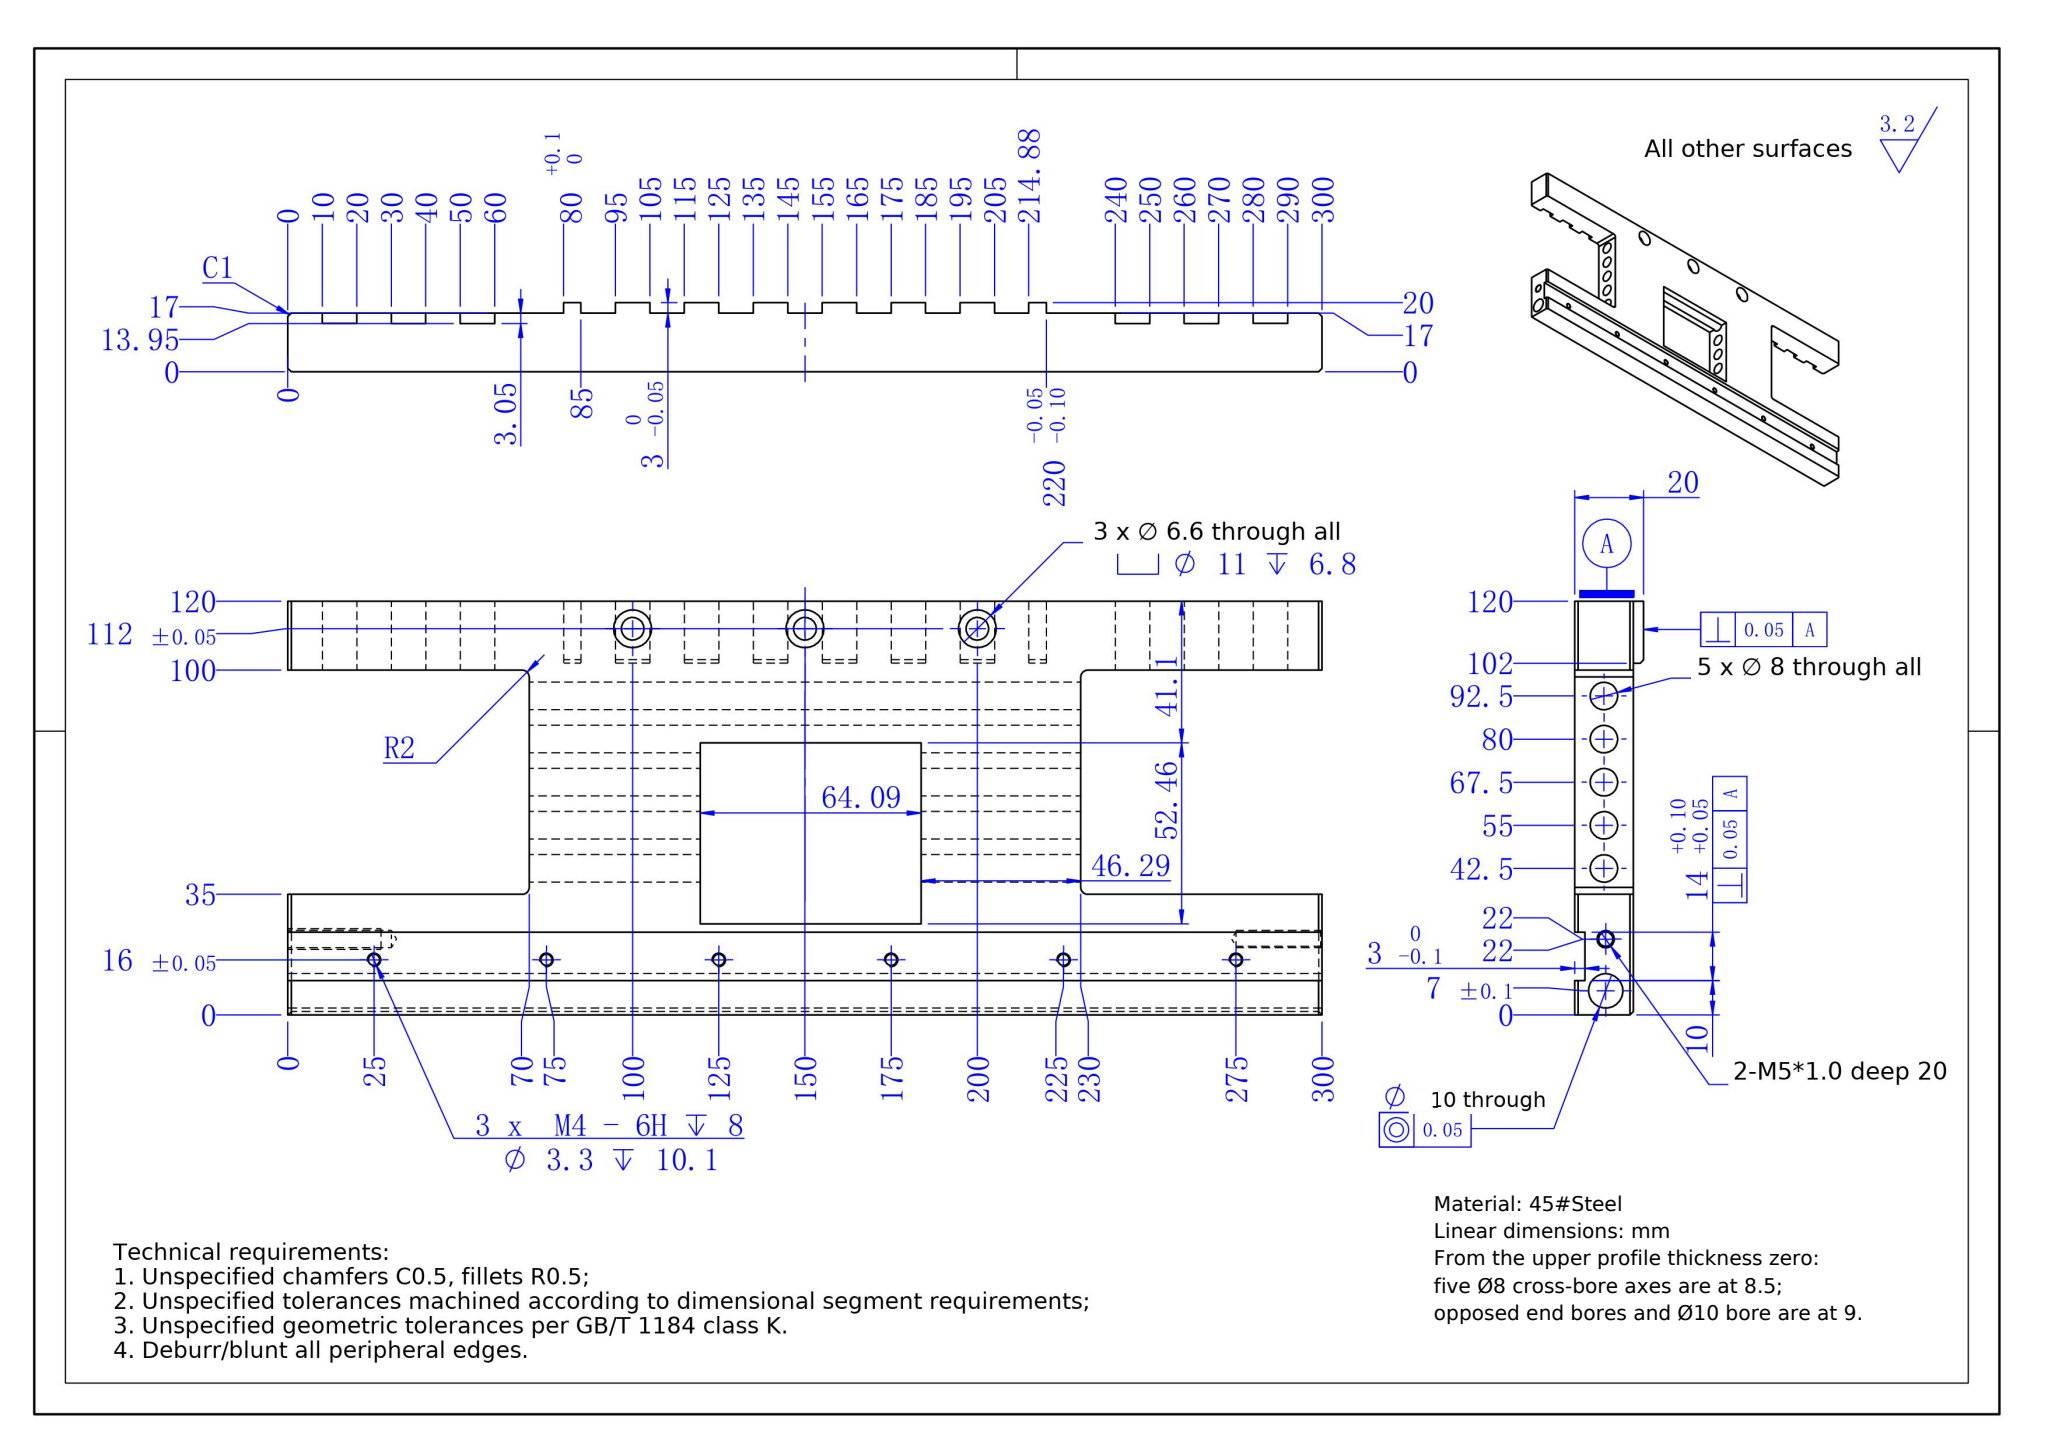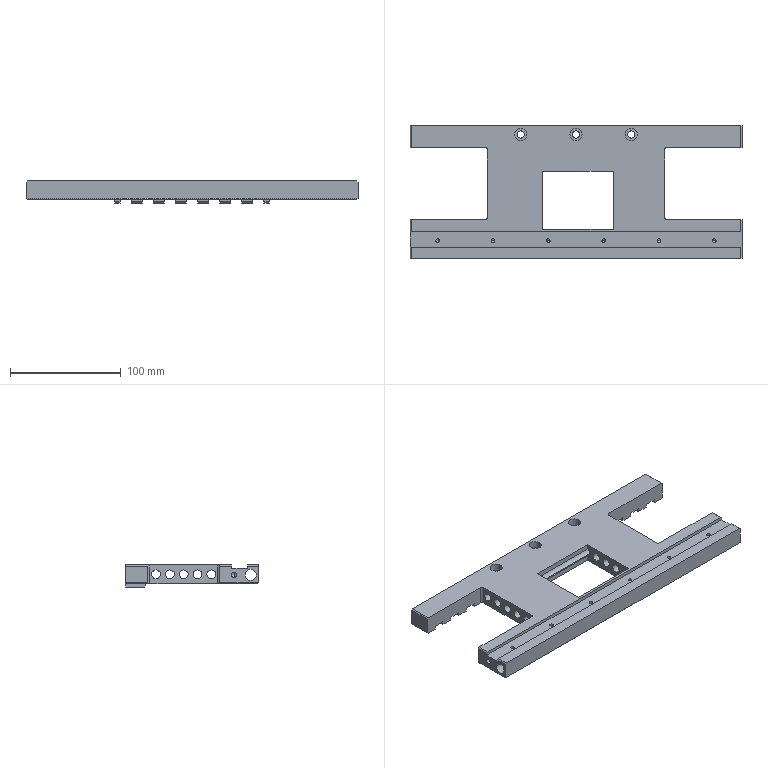Part | SolidWorks | mm | material 45#Steel | 1 solid | 169 faces | box 300 x 120 x 20 mm | volume 329731 mm3 | plane 101 | cylinder 50 | cone 18 | commonest cylinder face diameters 8 x16 3.3 x12 11 x6 6.6 x6 4 x4 5 x2 4.2 x2 10 x2
build123d program:
from build123d import *

# Parameters (mm, degrees)
SKETCH1_W                                         = 250
SKETCH1_H                                         = 120
EXTRUDE1_DEPTH                                    = 20
SKETCH8_W                                         = 3
SKETCH8_H                                         = 102
CUT_EXTRUDE7_DEPTH                                = 269.188
SKETCH15_W                                        = 17
SKETCH15_H                                        = 120
BOSS_EXTRUDE1_DEPTH                               = 25
SKETCH16_W                                        = 17
SKETCH16_H                                        = 120
BOSS_EXTRUDE2_DEPTH                               = 25
SKETCH17_R                                        = 5
CUT_EXTRUDE9_DEPTH                                = 316.317
M5_TAPPED_HOLE1_D                                 = 4.2
M5_TAPPED_HOLE1_DEPTH                             = 25
M5_TAPPED_HOLE1_CSINK_D                           = 5.05
M5_TAPPED_HOLE1_CSINK_ANGLE                       = 90
M5_TAPPED_HOLE1_TIP                               = 1.262
CHAMFER2_SIZE                                     = 3
CHAMFER3_SIZE                                     = 1
M6_TAPPED_HOLE2_D                                 = 5
M6_TAPPED_HOLE2_DEPTH                             = 30
M6_TAPPED_HOLE2_TIP                               = 1.502
CUT_EXTRUDE11_REACH                               = 274.855
SKETCH23_W                                        = 55
SKETCH23_H                                        = 18
CHAMFER5_SIZE                                     = 1
SKETCH24_W                                        = 3
SKETCH24_H                                        = 14
CUT_EXTRUDE12_DEPTH                               = 316.317
M4_TAPPED_HOLE1_AT_2_COUNT                        = 2
M4_TAPPED_HOLE1_AT_2_PITCH                        = 50
M4_TAPPED_HOLE1_AT_3_COUNT                        = 2
M4_TAPPED_HOLE1_AT_3_PITCH                        = 100
SKETCH27_W                                        = 70
SKETCH27_H                                        = 65
CUT_EXTRUDE13_DEPTH                               = 273.652
FILLET1_R                                         = 2
F_8_0_8_DIAMETER_HOLE1_D                          = 8
HOLE_SIZE_ACCORDING_TO_HEXAGON_SOCKET_D           = 6.6
HOLE_SIZE_ACCORDING_TO_HEXAGON_SOCKET_CBORE_D     = 11
HOLE_SIZE_ACCORDING_TO_HEXAGON_SOCKET_CBORE_DEPTH = 6.8
SKETCH32_W                                        = 10
SKETCH32_H                                        = 3
SKETCH32_H_2                                      = 3.046
CUT_EXTRUDE14_DEPTH                               = 20
CUT_EXTRUDE15_REACH                               = 284.533
SKETCH33_W                                        = 10
SKETCH33_H                                        = 3
SKETCH33_W_2                                      = 9.878
SKETCH34_W                                        = 64.093
SKETCH34_H                                        = 52.462
CUT_EXTRUDE16_DEPTH                               = 110


with BuildPart() as part:
    # Sketch1 → Extrude1 (new body)
    with BuildSketch(Plane.XY):
        with Locations((105, 35)):
            Rectangle(SKETCH1_W, SKETCH1_H)
    extrude(amount=EXTRUDE1_DEPTH)

    # Sketch8 → Cut-Extrude7 (cut, through all)
    with BuildSketch(Plane.ZY.offset(20)):
        with Locations((1.5, 26)):
            Rectangle(SKETCH8_W, SKETCH8_H)
    extrude(amount=-CUT_EXTRUDE7_DEPTH, mode=Mode.SUBTRACT)

    # Sketch15 → Boss-Extrude1 (add)
    with BuildSketch(Plane(origin=(230, 0, 0), x_dir=(0, 0, -1), z_dir=(1, 0, 0))):
        with Locations((-11.5, 35)):
            Rectangle(SKETCH15_W, SKETCH15_H)
    extrude(amount=BOSS_EXTRUDE1_DEPTH)

    # Sketch16 → Boss-Extrude2 (add)
    with BuildSketch(Plane.ZY.offset(20)):
        with Locations((11.5, 35)):
            Rectangle(SKETCH16_W, SKETCH16_H)
    extrude(amount=BOSS_EXTRUDE2_DEPTH)

    # Sketch17 → Cut-Extrude9 (cut, through all)
    with BuildSketch(Plane(origin=(255, 0, 0), x_dir=(0, 0, -1), z_dir=(1, 0, 0))):
        with Locations(Location((-11, -18, 0), (0, 0, 90))):
            Circle(SKETCH17_R)
    extrude(amount=-CUT_EXTRUDE9_DEPTH, mode=Mode.SUBTRACT)

    # M5 Tapped Hole1
    with Locations(Plane(origin=(255, 0, 0), x_dir=(0, 0, -1), z_dir=(1, 0, 0))):
        with Locations((-11, -3)):
            CounterSinkHole(M5_TAPPED_HOLE1_D / 2, M5_TAPPED_HOLE1_CSINK_D / 2, depth=M5_TAPPED_HOLE1_DEPTH, counter_sink_angle=M5_TAPPED_HOLE1_CSINK_ANGLE)
            with Locations((0, 0, -(M5_TAPPED_HOLE1_DEPTH + M5_TAPPED_HOLE1_TIP / 2))):  # 118° drill point
                Cone(0, M5_TAPPED_HOLE1_D / 2, M5_TAPPED_HOLE1_TIP, mode=Mode.SUBTRACT)

    # Chamfer2
    chamfer2_edges = [part.edges().sort_by_distance(p)[0] for p in [
        (230, 95, 1.5),
        (-20, 95, 1.5),
    ]]
    chamfer(chamfer2_edges, length=CHAMFER2_SIZE)

    # Chamfer3
    chamfer3_edges = [part.edges().sort_by_distance(p)[0] for p in [
        (105, 77, 0),
        (105, -25, 3),
    ]]
    chamfer(chamfer3_edges, length=CHAMFER3_SIZE)

    # M6 Tapped Hole2
    with Locations(Plane.ZY.offset(45)):
        with Locations((11, -3)):
            Hole(M6_TAPPED_HOLE2_D / 2, depth=M6_TAPPED_HOLE2_DEPTH)
            with Locations((0, 0, -(M6_TAPPED_HOLE2_DEPTH + M6_TAPPED_HOLE2_TIP / 2))):  # 118° drill point
                Cone(0, M6_TAPPED_HOLE2_D / 2, M6_TAPPED_HOLE2_TIP, mode=Mode.SUBTRACT)

    # Cut-Extrude11: up to this face of the body (flat: up to its plane)
    cut_extrude11_end = Plane(part.part.faces().sort_by_distance((105, 28.235, 3))[0])
    # Sketch23 → Cut-Extrude11 (cut, up to the picked face)
    with BuildSketch(Plane(origin=(0, 0, 0), x_dir=(-1, 0, 0), z_dir=(0, 0, -1)), mode=Mode.PRIVATE) as cut_extrude11_sk1:
        with Locations((-202.5, 86)):
            Rectangle(SKETCH23_W, SKETCH23_H)
    cut_extrude11_tool1 = split(extrude(cut_extrude11_sk1.sketch, amount=-CUT_EXTRUDE11_REACH, mode=Mode.PRIVATE), bisect_by=cut_extrude11_end, keep=Keep.BOTH, mode=Mode.PRIVATE)
    # Sketch23 → Cut-Extrude11 (cut, up to the picked face)
    with BuildSketch(Plane(origin=(0, 0, 0), x_dir=(-1, 0, 0), z_dir=(0, 0, -1)), mode=Mode.PRIVATE) as cut_extrude11_sk2:
        with Locations((-7.5, 86)):
            Rectangle(SKETCH23_W, SKETCH23_H)
    cut_extrude11_tool2 = split(extrude(cut_extrude11_sk2.sketch, amount=-CUT_EXTRUDE11_REACH, mode=Mode.PRIVATE), bisect_by=cut_extrude11_end, keep=Keep.BOTH, mode=Mode.PRIVATE)
    add(cut_extrude11_tool1.solids().sort_by(Axis((202.5, 86, 0), (0, 0, 1)))[0], mode=Mode.SUBTRACT)
    add(cut_extrude11_tool2.solids().sort_by(Axis((7.5, 86, 0), (0, 0, 1)))[0], mode=Mode.SUBTRACT)

    # Chamfer5
    chamfer5_edges = [part.edges().sort_by_distance(p)[0] for p in [
        (-45, 35, 20),
        (-45, 35.5, 3),
        (255, 35, 20),
        (255, 35.5, 3),
    ]]
    chamfer(chamfer5_edges, length=CHAMFER5_SIZE)

    # Sketch24 → Cut-Extrude12 (cut, through all)
    with BuildSketch(Plane.ZY.offset(45)):
        with Locations((18.5, -8)):
            Rectangle(SKETCH24_W, SKETCH24_H)
    extrude(amount=-CUT_EXTRUDE12_DEPTH, mode=Mode.SUBTRACT)

    # Sketch26 → M4 Tapped Hole1 (revolve, cut)
    with BuildSketch(Plane(origin=(-20, -9, 17), x_dir=(0, -1, 0), z_dir=(1, 0, 0))):
        Polygon((0, 0), (0, 11.091), (1.65, 10.1), (1.65, 0), align=None)
    m4_tapped_hole1 = revolve(axis=Axis((-20, -9, 23.35), (0, 0, -1)), mode=Mode.SUBTRACT)

    # M4 Tapped Hole1 at 2: M4 Tapped Hole1 ×2
    with Locations(*[(i * M4_TAPPED_HOLE1_AT_2_PITCH, 0, 0) for i in range(1, M4_TAPPED_HOLE1_AT_2_COUNT)]):
        add(m4_tapped_hole1, mode=Mode.SUBTRACT)

    # M4 Tapped Hole1 at 3: M4 Tapped Hole1 ×2
    with Locations(*[(i * M4_TAPPED_HOLE1_AT_3_PITCH, 0, 0) for i in range(1, M4_TAPPED_HOLE1_AT_3_COUNT)]):
        add(m4_tapped_hole1, mode=Mode.SUBTRACT)

    # Sketch27 → Cut-Extrude13 (cut, through all)
    with BuildSketch(Plane(origin=(0, 0, 3), x_dir=(-1, 0, 0), z_dir=(0, 0, -1))):
        with Locations((-220, 42.5)):
            Rectangle(SKETCH27_W, SKETCH27_H)
    cut_extrude13 = extrude(amount=-CUT_EXTRUDE13_DEPTH, mode=Mode.SUBTRACT)

    # Mirror1: Cut-Extrude13 across plane
    add(cut_extrude13.mirror(Plane(origin=(105, 0, 0), x_dir=(0, 0, 1), z_dir=(1, 0, 0))), mode=Mode.SUBTRACT)

    # Fillet1
    fillet1_edges = [part.edges().sort_by_distance(p)[0] for p in [
        (185, 75, 11.5),
        (185, 10, 11.5),
        (25, 10, 11.5),
        (25, 75, 11.5),
    ]]
    fillet(fillet1_edges, radius=FILLET1_R)

    # 8.0 _8_ Diameter Hole1 (through all)
    with Locations(Plane(origin=(185, 0, 0), x_dir=(0, 0, -1), z_dir=(1, 0, 0))):
        with Locations((-11.5, 67.5), (-11.5, 42.5), (-11.5, 17.5), (-11.5, 55), (-11.5, 30)):
            Hole(F_8_0_8_DIAMETER_HOLE1_D / 2)

    # Hole Size _According to_ Hexagon Socket (through all)
    with Locations(Plane.XY.offset(20)):
        with Locations((155, 87), (55, 87), (105, 87)):
            CounterBoreHole(HOLE_SIZE_ACCORDING_TO_HEXAGON_SOCKET_D / 2, HOLE_SIZE_ACCORDING_TO_HEXAGON_SOCKET_CBORE_D / 2, HOLE_SIZE_ACCORDING_TO_HEXAGON_SOCKET_CBORE_DEPTH)

    # Sketch32 → Cut-Extrude14 (cut)
    with BuildSketch(Plane(origin=(0, 95, 0), x_dir=(1, 0, 0), z_dir=(0, 1, 0))):
        with Locations((-30, -4.5)):
            Rectangle(SKETCH32_W, SKETCH32_H)
        with Locations((-10, -4.523)):
            Rectangle(SKETCH32_W, SKETCH32_H_2)
        with Locations((10, -4.523)):
            Rectangle(SKETCH32_W, SKETCH32_H_2)
    cut_extrude14 = extrude(amount=-CUT_EXTRUDE14_DEPTH, mode=Mode.SUBTRACT)

    # Mirror2: Cut-Extrude14 across plane
    add(cut_extrude14.mirror(Plane(origin=(105, 0, 0), x_dir=(0, 0, 1), z_dir=(1, 0, 0))), mode=Mode.SUBTRACT)

    # Cut-Extrude15: up to this face of the body (flat: up to its plane)
    cut_extrude15_end = Plane(part.part.faces().sort_by_distance((105, 77, 2))[0])
    # Sketch33 → Cut-Extrude15 (cut, up to the picked face)
    with BuildSketch(Plane(origin=(0, 95, 0), x_dir=(1, 0, 0), z_dir=(0, 1, 0)), mode=Mode.PRIVATE) as cut_extrude15_sk1:
        with Locations((45, -1.5)):
            Rectangle(SKETCH33_W, SKETCH33_H)
    cut_extrude15_tool1 = split(extrude(cut_extrude15_sk1.sketch, amount=-CUT_EXTRUDE15_REACH, mode=Mode.PRIVATE), bisect_by=cut_extrude15_end, keep=Keep.BOTH, mode=Mode.PRIVATE)
    # Sketch33 → Cut-Extrude15 (cut, up to the picked face)
    with BuildSketch(Plane(origin=(0, 95, 0), x_dir=(1, 0, 0), z_dir=(0, 1, 0)), mode=Mode.PRIVATE) as cut_extrude15_sk2:
        with Locations((65, -1.5)):
            Rectangle(SKETCH33_W, SKETCH33_H)
    cut_extrude15_tool2 = split(extrude(cut_extrude15_sk2.sketch, amount=-CUT_EXTRUDE15_REACH, mode=Mode.PRIVATE), bisect_by=cut_extrude15_end, keep=Keep.BOTH, mode=Mode.PRIVATE)
    # Sketch33 → Cut-Extrude15 (cut, up to the picked face)
    with BuildSketch(Plane(origin=(0, 95, 0), x_dir=(1, 0, 0), z_dir=(0, 1, 0)), mode=Mode.PRIVATE) as cut_extrude15_sk3:
        with Locations((85, -1.5)):
            Rectangle(SKETCH33_W, SKETCH33_H)
    cut_extrude15_tool3 = split(extrude(cut_extrude15_sk3.sketch, amount=-CUT_EXTRUDE15_REACH, mode=Mode.PRIVATE), bisect_by=cut_extrude15_end, keep=Keep.BOTH, mode=Mode.PRIVATE)
    # Sketch33 → Cut-Extrude15 (cut, up to the picked face)
    with BuildSketch(Plane(origin=(0, 95, 0), x_dir=(1, 0, 0), z_dir=(0, 1, 0)), mode=Mode.PRIVATE) as cut_extrude15_sk4:
        with Locations((105, -1.5)):
            Rectangle(SKETCH33_W, SKETCH33_H)
    cut_extrude15_tool4 = split(extrude(cut_extrude15_sk4.sketch, amount=-CUT_EXTRUDE15_REACH, mode=Mode.PRIVATE), bisect_by=cut_extrude15_end, keep=Keep.BOTH, mode=Mode.PRIVATE)
    # Sketch33 → Cut-Extrude15 (cut, up to the picked face)
    with BuildSketch(Plane(origin=(0, 95, 0), x_dir=(1, 0, 0), z_dir=(0, 1, 0)), mode=Mode.PRIVATE) as cut_extrude15_sk5:
        with Locations((125, -1.5)):
            Rectangle(SKETCH33_W, SKETCH33_H)
    cut_extrude15_tool5 = split(extrude(cut_extrude15_sk5.sketch, amount=-CUT_EXTRUDE15_REACH, mode=Mode.PRIVATE), bisect_by=cut_extrude15_end, keep=Keep.BOTH, mode=Mode.PRIVATE)
    # Sketch33 → Cut-Extrude15 (cut, up to the picked face)
    with BuildSketch(Plane(origin=(0, 95, 0), x_dir=(1, 0, 0), z_dir=(0, 1, 0)), mode=Mode.PRIVATE) as cut_extrude15_sk6:
        with Locations((145, -1.5)):
            Rectangle(SKETCH33_W, SKETCH33_H)
    cut_extrude15_tool6 = split(extrude(cut_extrude15_sk6.sketch, amount=-CUT_EXTRUDE15_REACH, mode=Mode.PRIVATE), bisect_by=cut_extrude15_end, keep=Keep.BOTH, mode=Mode.PRIVATE)
    # Sketch33 → Cut-Extrude15 (cut, up to the picked face)
    with BuildSketch(Plane(origin=(0, 95, 0), x_dir=(1, 0, 0), z_dir=(0, 1, 0)), mode=Mode.PRIVATE) as cut_extrude15_sk7:
        with Locations((164.939, -1.5)):
            Rectangle(SKETCH33_W_2, SKETCH33_H)
    cut_extrude15_tool7 = split(extrude(cut_extrude15_sk7.sketch, amount=-CUT_EXTRUDE15_REACH, mode=Mode.PRIVATE), bisect_by=cut_extrude15_end, keep=Keep.BOTH, mode=Mode.PRIVATE)
    add(cut_extrude15_tool1.solids().sort_by(Axis((45, 95, 1.5), (0, -1, 0)))[0], mode=Mode.SUBTRACT)
    add(cut_extrude15_tool2.solids().sort_by(Axis((65, 95, 1.5), (0, -1, 0)))[0], mode=Mode.SUBTRACT)
    add(cut_extrude15_tool3.solids().sort_by(Axis((85, 95, 1.5), (0, -1, 0)))[0], mode=Mode.SUBTRACT)
    add(cut_extrude15_tool4.solids().sort_by(Axis((105, 95, 1.5), (0, -1, 0)))[0], mode=Mode.SUBTRACT)
    add(cut_extrude15_tool5.solids().sort_by(Axis((125, 95, 1.5), (0, -1, 0)))[0], mode=Mode.SUBTRACT)
    add(cut_extrude15_tool6.solids().sort_by(Axis((145, 95, 1.5), (0, -1, 0)))[0], mode=Mode.SUBTRACT)
    add(cut_extrude15_tool7.solids().sort_by(Axis((164.939, 95, 1.5), (0, -1, 0)))[0], mode=Mode.SUBTRACT)

    # Mirror3: M4 Tapped Hole1 across plane
    add(m4_tapped_hole1.mirror(Plane(origin=(105, 0, 0), x_dir=(0, 0, 1), z_dir=(1, 0, 0))), mode=Mode.SUBTRACT)

    # Mirror3 copy 1 sketch → Mirror3 copy 1 (revolve, cut)
    with BuildSketch(Plane(origin=(180, -9, 17), x_dir=(0, -1, 0), z_dir=(-1, 0, 0))):
        Polygon((0, 0), (0, -11.091), (1.65, -10.1), (1.65, 0), align=None)
    revolve(axis=Axis((180, -9, 23.35), (0, 0, 1)), mode=Mode.SUBTRACT)

    # Mirror3 copy 2 sketch → Mirror3 copy 2 (revolve, cut)
    with BuildSketch(Plane(origin=(130, -9, 17), x_dir=(0, -1, 0), z_dir=(-1, 0, 0))):
        Polygon((0, 0), (0, -11.091), (1.65, -10.1), (1.65, 0), align=None)
    revolve(axis=Axis((130, -9, 23.35), (0, 0, 1)), mode=Mode.SUBTRACT)

    # Sketch34 → Cut-Extrude16 (cut)
    with BuildSketch(Plane(origin=(0, 0, 3), x_dir=(-1, 0, 0), z_dir=(0, 0, -1))):
        with Locations((-106.662, 27.666)):
            Rectangle(SKETCH34_W, SKETCH34_H)
    extrude(amount=-CUT_EXTRUDE16_DEPTH, mode=Mode.SUBTRACT)


solid = part.part